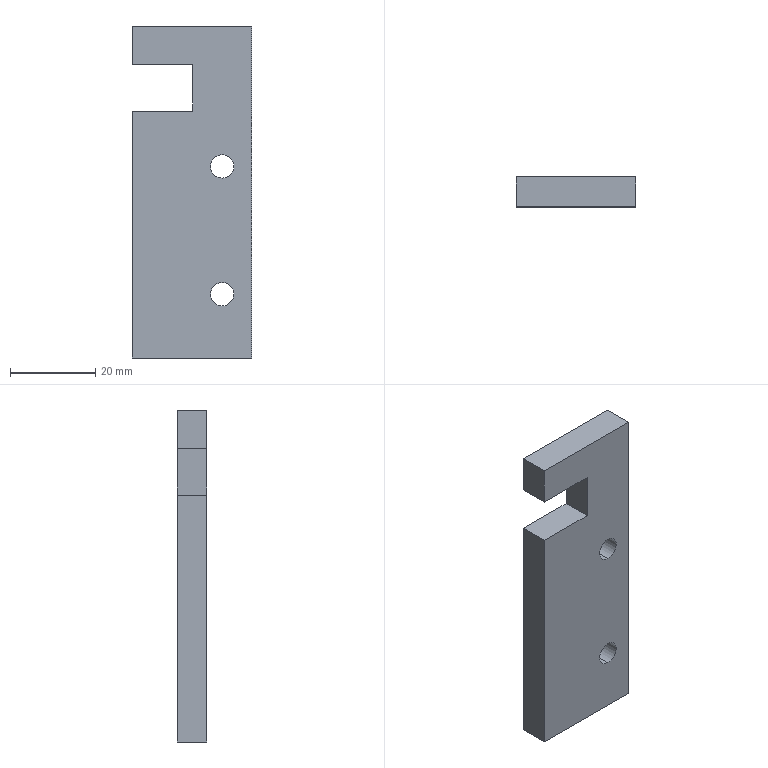Component | SolidWorks | PointedHeadDispensingCoverPlateA-1 | 1 solid | 14 faces | box 28 x 7 x 78 mm | volume 13862 mm3 | plane 10 | cylinder 4 | commonest cylinder face diameters 5.5 x4
build123d program:
from build123d import *

# Parameters (mm, degrees)
SKETCH1_W                  = 28
SKETCH1_H                  = 78
EXTRUDE1_DEPTH             = 7
SKETCH2_W                  = 14.2
SKETCH2_H                  = 11
CUT_EXTRUDE1_DEPTH         = 84.169
F_5_5_5_5_DIAMETER_HOLE1_D = 5.5


with BuildPart() as part:
    # Sketch1 → Extrude1 (new body)
    with BuildSketch(Plane(origin=(0, 0, 0), x_dir=(1, 0, 0), z_dir=(0, 1, 0))):
        with Locations((14, -39)):
            Rectangle(SKETCH1_W, SKETCH1_H)
    extrude(amount=EXTRUDE1_DEPTH)

    # Sketch2 → Cut-Extrude1 (cut, through all)
    with BuildSketch(Plane(origin=(0, 7, 0), x_dir=(1, 0, 0), z_dir=(0, 1, 0))):
        with Locations((7.1, -63.5)):
            Rectangle(SKETCH2_W, SKETCH2_H)
    extrude(amount=-CUT_EXTRUDE1_DEPTH, mode=Mode.SUBTRACT)

    # 5.5 _5.5_ Diameter Hole1 (through all)
    with Locations(Plane(origin=(0, 7, 0), x_dir=(-1, 0, 0), z_dir=(0, 1, 0))):
        with Locations((-21.1, 45), (-21.1, 15)):
            Hole(F_5_5_5_5_DIAMETER_HOLE1_D / 2)


solid = part.part

# Placed as in the assembly
solid = solid.moved(Location((10.917, 82.372, -117.387), (0, 0, 0)))
STEP:
#1=COLOUR_RGB('',0.7922,0.8196,0.9333);
#2=FILL_AREA_STYLE_COLOUR('',#1);
#3=FILL_AREA_STYLE('',(#2));
#4=SURFACE_STYLE_FILL_AREA(#3);
#5=SURFACE_SIDE_STYLE('',(#4));
#6=SURFACE_STYLE_USAGE(.BOTH.,#5);
#7=PRESENTATION_STYLE_ASSIGNMENT((#6));
#8=CARTESIAN_POINT('',(1.261,3.243,-2.958));
#9=VERTEX_POINT('',#8);
#10=CARTESIAN_POINT('',(1.261,3.243,-2.742));
#11=VERTEX_POINT('',#10);
#12=CARTESIAN_POINT('',(1.261,3.243,-2.85));
#13=DIRECTION('',(0.,1.,0.));
#14=DIRECTION('',(0.,0.,1.));
#15=AXIS2_PLACEMENT_3D('',#12,#13,#14);
#16=CIRCLE('',#15,0.1083);
#17=EDGE_CURVE('',#9,#11,#16,.T.);
#18=ORIENTED_EDGE('',*,*,#17,.F.);
#19=CARTESIAN_POINT('',(1.261,3.519,-2.958));
#20=VERTEX_POINT('',#19);
#21=CARTESIAN_POINT('',(1.261,3.519,-2.958));
#22=DIRECTION('',(0.,1.,0.));
#23=VECTOR('',#22,39.37);
#24=LINE('',#21,#23);
#25=EDGE_CURVE('',#9,#20,#24,.T.);
#26=ORIENTED_EDGE('',*,*,#25,.T.);
#27=CARTESIAN_POINT('',(1.261,3.519,-2.742));
#28=VERTEX_POINT('',#27);
#29=CARTESIAN_POINT('',(1.261,3.519,-2.85));
#30=DIRECTION('',(0.,1.,0.));
#31=DIRECTION('',(0.,0.,1.));
#32=AXIS2_PLACEMENT_3D('',#29,#30,#31);
#33=CIRCLE('',#32,0.1083);
#34=EDGE_CURVE('',#20,#28,#33,.T.);
#35=ORIENTED_EDGE('',*,*,#34,.T.);
#36=CARTESIAN_POINT('',(1.261,3.519,-2.742));
#37=DIRECTION('',(0.,1.,0.));
#38=VECTOR('',#37,39.37);
#39=LINE('',#36,#38);
#40=EDGE_CURVE('',#11,#28,#39,.T.);
#41=ORIENTED_EDGE('',*,*,#40,.F.);
#42=EDGE_LOOP('',(#18,#26,#35,#41));
#43=FACE_OUTER_BOUND('',#42,.T.);
#44=CARTESIAN_POINT('',(1.261,3.519,-2.85));
#45=DIRECTION('',(0.,1.,0.));
#46=DIRECTION('',(0.,0.,1.));
#47=AXIS2_PLACEMENT_3D('',#44,#45,#46);
#48=CYLINDRICAL_SURFACE('',#47,0.1083);
#49=ADVANCED_FACE('',(#43),#48,.F.);
#50=CARTESIAN_POINT('',(1.261,3.243,-4.139));
#51=VERTEX_POINT('',#50);
#52=CARTESIAN_POINT('',(1.261,3.243,-3.923));
#53=VERTEX_POINT('',#52);
#54=CARTESIAN_POINT('',(1.261,3.243,-4.031));
#55=DIRECTION('',(0.,1.,0.));
#56=DIRECTION('',(0.,0.,1.));
#57=AXIS2_PLACEMENT_3D('',#54,#55,#56);
#58=CIRCLE('',#57,0.1083);
#59=EDGE_CURVE('',#51,#53,#58,.T.);
#60=ORIENTED_EDGE('',*,*,#59,.F.);
#61=CARTESIAN_POINT('',(1.261,3.519,-4.139));
#62=VERTEX_POINT('',#61);
#63=CARTESIAN_POINT('',(1.261,3.519,-4.139));
#64=DIRECTION('',(0.,1.,0.));
#65=VECTOR('',#64,39.37);
#66=LINE('',#63,#65);
#67=EDGE_CURVE('',#51,#62,#66,.T.);
#68=ORIENTED_EDGE('',*,*,#67,.T.);
#69=CARTESIAN_POINT('',(1.261,3.519,-3.923));
#70=VERTEX_POINT('',#69);
#71=CARTESIAN_POINT('',(1.261,3.519,-4.031));
#72=DIRECTION('',(0.,1.,0.));
#73=DIRECTION('',(0.,0.,1.));
#74=AXIS2_PLACEMENT_3D('',#71,#72,#73);
#75=CIRCLE('',#74,0.1083);
#76=EDGE_CURVE('',#62,#70,#75,.T.);
#77=ORIENTED_EDGE('',*,*,#76,.T.);
#78=CARTESIAN_POINT('',(1.261,3.519,-3.923));
#79=DIRECTION('',(0.,1.,0.));
#80=VECTOR('',#79,39.37);
#81=LINE('',#78,#80);
#82=EDGE_CURVE('',#53,#70,#81,.T.);
#83=ORIENTED_EDGE('',*,*,#82,.F.);
#84=EDGE_LOOP('',(#60,#68,#77,#83));
#85=FACE_OUTER_BOUND('',#84,.T.);
#86=CARTESIAN_POINT('',(1.261,3.519,-4.031));
#87=DIRECTION('',(0.,1.,0.));
#88=DIRECTION('',(0.,0.,1.));
#89=AXIS2_PLACEMENT_3D('',#86,#87,#88);
#90=CYLINDRICAL_SURFACE('',#89,0.1083);
#91=ADVANCED_FACE('',(#85),#90,.F.);
#92=CARTESIAN_POINT('',(0.4298,3.243,-4.622));
#93=VERTEX_POINT('',#92);
#94=CARTESIAN_POINT('',(0.4298,3.243,-2.338));
#95=VERTEX_POINT('',#94);
#96=CARTESIAN_POINT('',(0.4298,3.243,-4.622));
#97=DIRECTION('',(0.,0.,1.));
#98=VECTOR('',#97,39.37);
#99=LINE('',#96,#98);
#100=EDGE_CURVE('',#93,#95,#99,.T.);
#101=ORIENTED_EDGE('',*,*,#100,.T.);
#102=CARTESIAN_POINT('',(0.4298,3.519,-2.338));
#103=VERTEX_POINT('',#102);
#104=CARTESIAN_POINT('',(0.4298,3.243,-2.338));
#105=DIRECTION('',(0.,1.,0.));
#106=VECTOR('',#105,39.37);
#107=LINE('',#104,#106);
#108=EDGE_CURVE('',#95,#103,#107,.T.);
#109=ORIENTED_EDGE('',*,*,#108,.T.);
#110=CARTESIAN_POINT('',(0.4298,3.519,-4.622));
#111=VERTEX_POINT('',#110);
#112=CARTESIAN_POINT('',(0.4298,3.519,-4.622));
#113=DIRECTION('',(0.,0.,1.));
#114=VECTOR('',#113,39.37);
#115=LINE('',#112,#114);
#116=EDGE_CURVE('',#111,#103,#115,.T.);
#117=ORIENTED_EDGE('',*,*,#116,.F.);
#118=CARTESIAN_POINT('',(0.4298,3.519,-4.622));
#119=DIRECTION('',(0.,-1.,0.));
#120=VECTOR('',#119,39.37);
#121=LINE('',#118,#120);
#122=EDGE_CURVE('',#111,#93,#121,.T.);
#123=ORIENTED_EDGE('',*,*,#122,.T.);
#124=EDGE_LOOP('',(#101,#109,#117,#123));
#125=FACE_OUTER_BOUND('',#124,.T.);
#126=CARTESIAN_POINT('',(0.4298,3.519,-4.622));
#127=DIRECTION('',(1.,0.,-0.));
#128=DIRECTION('',(-0.,0.,-1.));
#129=AXIS2_PLACEMENT_3D('',#126,#127,#128);
#130=PLANE('',#129);
#131=ADVANCED_FACE('',(#125),#130,.F.);
#132=CARTESIAN_POINT('',(0.4298,3.519,-1.905));
#133=VERTEX_POINT('',#132);
#134=CARTESIAN_POINT('',(0.4298,3.519,-1.551));
#135=VERTEX_POINT('',#134);
#136=CARTESIAN_POINT('',(0.4298,3.519,-4.622));
#137=DIRECTION('',(0.,0.,1.));
#138=VECTOR('',#137,39.37);
#139=LINE('',#136,#138);
#140=EDGE_CURVE('',#133,#135,#139,.T.);
#141=ORIENTED_EDGE('',*,*,#140,.F.);
#142=CARTESIAN_POINT('',(0.4298,3.243,-1.905));
#143=VERTEX_POINT('',#142);
#144=CARTESIAN_POINT('',(0.4298,3.243,-1.905));
#145=DIRECTION('',(0.,1.,0.));
#146=VECTOR('',#145,39.37);
#147=LINE('',#144,#146);
#148=EDGE_CURVE('',#143,#133,#147,.T.);
#149=ORIENTED_EDGE('',*,*,#148,.F.);
#150=CARTESIAN_POINT('',(0.4298,3.243,-1.551));
#151=VERTEX_POINT('',#150);
#152=CARTESIAN_POINT('',(0.4298,3.243,-4.622));
#153=DIRECTION('',(0.,0.,1.));
#154=VECTOR('',#153,39.37);
#155=LINE('',#152,#154);
#156=EDGE_CURVE('',#143,#151,#155,.T.);
#157=ORIENTED_EDGE('',*,*,#156,.T.);
#158=CARTESIAN_POINT('',(0.4298,3.519,-1.551));
#159=DIRECTION('',(0.,-1.,0.));
#160=VECTOR('',#159,39.37);
#161=LINE('',#158,#160);
#162=EDGE_CURVE('',#135,#151,#161,.T.);
#163=ORIENTED_EDGE('',*,*,#162,.F.);
#164=EDGE_LOOP('',(#141,#149,#157,#163));
#165=FACE_OUTER_BOUND('',#164,.T.);
#166=CARTESIAN_POINT('',(0.4298,3.519,-4.622));
#167=DIRECTION('',(1.,0.,-0.));
#168=DIRECTION('',(-0.,0.,-1.));
#169=AXIS2_PLACEMENT_3D('',#166,#167,#168);
#170=PLANE('',#169);
#171=ADVANCED_FACE('',(#165),#170,.F.);
#172=CARTESIAN_POINT('',(1.532,3.243,-1.551));
#173=VERTEX_POINT('',#172);
#174=CARTESIAN_POINT('',(0.4298,3.243,-1.551));
#175=DIRECTION('',(1.,0.,0.));
#176=VECTOR('',#175,39.37);
#177=LINE('',#174,#176);
#178=EDGE_CURVE('',#151,#173,#177,.T.);
#179=ORIENTED_EDGE('',*,*,#178,.T.);
#180=CARTESIAN_POINT('',(1.532,3.519,-1.551));
#181=VERTEX_POINT('',#180);
#182=CARTESIAN_POINT('',(1.532,3.519,-1.551));
#183=DIRECTION('',(0.,-1.,0.));
#184=VECTOR('',#183,39.37);
#185=LINE('',#182,#184);
#186=EDGE_CURVE('',#181,#173,#185,.T.);
#187=ORIENTED_EDGE('',*,*,#186,.F.);
#188=CARTESIAN_POINT('',(0.4298,3.519,-1.551));
#189=DIRECTION('',(1.,0.,0.));
#190=VECTOR('',#189,39.37);
#191=LINE('',#188,#190);
#192=EDGE_CURVE('',#135,#181,#191,.T.);
#193=ORIENTED_EDGE('',*,*,#192,.F.);
#194=ORIENTED_EDGE('',*,*,#162,.T.);
#195=EDGE_LOOP('',(#179,#187,#193,#194));
#196=FACE_OUTER_BOUND('',#195,.T.);
#197=CARTESIAN_POINT('',(0.4298,3.519,-1.551));
#198=DIRECTION('',(0.,0.,-1.));
#199=DIRECTION('',(-1.,0.,0.));
#200=AXIS2_PLACEMENT_3D('',#197,#198,#199);
#201=PLANE('',#200);
#202=ADVANCED_FACE('',(#196),#201,.F.);
#203=CARTESIAN_POINT('',(1.532,3.243,-4.622));
#204=VERTEX_POINT('',#203);
#205=CARTESIAN_POINT('',(1.532,3.243,-4.622));
#206=DIRECTION('',(-0.,0.,-1.));
#207=VECTOR('',#206,39.37);
#208=LINE('',#205,#207);
#209=EDGE_CURVE('',#173,#204,#208,.T.);
#210=ORIENTED_EDGE('',*,*,#209,.T.);
#211=CARTESIAN_POINT('',(1.532,3.519,-4.622));
#212=VERTEX_POINT('',#211);
#213=CARTESIAN_POINT('',(1.532,3.519,-4.622));
#214=DIRECTION('',(0.,-1.,0.));
#215=VECTOR('',#214,39.37);
#216=LINE('',#213,#215);
#217=EDGE_CURVE('',#212,#204,#216,.T.);
#218=ORIENTED_EDGE('',*,*,#217,.F.);
#219=CARTESIAN_POINT('',(1.532,3.519,-4.622));
#220=DIRECTION('',(-0.,0.,-1.));
#221=VECTOR('',#220,39.37);
#222=LINE('',#219,#221);
#223=EDGE_CURVE('',#181,#212,#222,.T.);
#224=ORIENTED_EDGE('',*,*,#223,.F.);
#225=ORIENTED_EDGE('',*,*,#186,.T.);
#226=EDGE_LOOP('',(#210,#218,#224,#225));
#227=FACE_OUTER_BOUND('',#226,.T.);
#228=CARTESIAN_POINT('',(1.532,3.519,-4.622));
#229=DIRECTION('',(-1.,0.,0.));
#230=DIRECTION('',(0.,0.,1.));
#231=AXIS2_PLACEMENT_3D('',#228,#229,#230);
#232=PLANE('',#231);
#233=ADVANCED_FACE('',(#227),#232,.F.);
#234=CARTESIAN_POINT('',(0.4298,3.243,-4.622));
#235=DIRECTION('',(-1.,0.,0.));
#236=VECTOR('',#235,39.37);
#237=LINE('',#234,#236);
#238=EDGE_CURVE('',#204,#93,#237,.T.);
#239=ORIENTED_EDGE('',*,*,#238,.T.);
#240=ORIENTED_EDGE('',*,*,#122,.F.);
#241=CARTESIAN_POINT('',(0.4298,3.519,-4.622));
#242=DIRECTION('',(-1.,0.,0.));
#243=VECTOR('',#242,39.37);
#244=LINE('',#241,#243);
#245=EDGE_CURVE('',#212,#111,#244,.T.);
#246=ORIENTED_EDGE('',*,*,#245,.F.);
#247=ORIENTED_EDGE('',*,*,#217,.T.);
#248=EDGE_LOOP('',(#239,#240,#246,#247));
#249=FACE_OUTER_BOUND('',#248,.T.);
#250=CARTESIAN_POINT('',(0.4298,3.519,-4.622));
#251=DIRECTION('',(0.,0.,1.));
#252=DIRECTION('',(1.,0.,0.));
#253=AXIS2_PLACEMENT_3D('',#250,#251,#252);
#254=PLANE('',#253);
#255=ADVANCED_FACE('',(#249),#254,.F.);
#256=CARTESIAN_POINT('',(1.261,3.519,-2.85));
#257=DIRECTION('',(0.,1.,0.));
#258=DIRECTION('',(0.,0.,1.));
#259=AXIS2_PLACEMENT_3D('',#256,#257,#258);
#260=CIRCLE('',#259,0.1083);
#261=EDGE_CURVE('',#28,#20,#260,.T.);
#262=ORIENTED_EDGE('',*,*,#261,.F.);
#263=ORIENTED_EDGE('',*,*,#34,.F.);
#264=EDGE_LOOP('',(#262,#263));
#265=FACE_BOUND('',#264,.T.);
#266=CARTESIAN_POINT('',(1.261,3.519,-4.031));
#267=DIRECTION('',(0.,1.,0.));
#268=DIRECTION('',(0.,0.,1.));
#269=AXIS2_PLACEMENT_3D('',#266,#267,#268);
#270=CIRCLE('',#269,0.1083);
#271=EDGE_CURVE('',#70,#62,#270,.T.);
#272=ORIENTED_EDGE('',*,*,#271,.F.);
#273=ORIENTED_EDGE('',*,*,#76,.F.);
#274=EDGE_LOOP('',(#272,#273));
#275=FACE_BOUND('',#274,.T.);
#276=CARTESIAN_POINT('',(0.9889,3.519,-2.338));
#277=VERTEX_POINT('',#276);
#278=CARTESIAN_POINT('',(0.4298,3.519,-2.338));
#279=DIRECTION('',(-1.,0.,-0.));
#280=VECTOR('',#279,39.37);
#281=LINE('',#278,#280);
#282=EDGE_CURVE('',#277,#103,#281,.T.);
#283=ORIENTED_EDGE('',*,*,#282,.F.);
#284=CARTESIAN_POINT('',(0.9889,3.519,-1.905));
#285=VERTEX_POINT('',#284);
#286=CARTESIAN_POINT('',(0.9889,3.519,-1.905));
#287=DIRECTION('',(0.,0.,-1.));
#288=VECTOR('',#287,39.37);
#289=LINE('',#286,#288);
#290=EDGE_CURVE('',#285,#277,#289,.T.);
#291=ORIENTED_EDGE('',*,*,#290,.F.);
#292=CARTESIAN_POINT('',(0.4298,3.519,-1.905));
#293=DIRECTION('',(1.,0.,0.));
#294=VECTOR('',#293,39.37);
#295=LINE('',#292,#294);
#296=EDGE_CURVE('',#133,#285,#295,.T.);
#297=ORIENTED_EDGE('',*,*,#296,.F.);
#298=ORIENTED_EDGE('',*,*,#140,.T.);
#299=ORIENTED_EDGE('',*,*,#192,.T.);
#300=ORIENTED_EDGE('',*,*,#223,.T.);
#301=ORIENTED_EDGE('',*,*,#245,.T.);
#302=ORIENTED_EDGE('',*,*,#116,.T.);
#303=EDGE_LOOP('',(#283,#291,#297,#298,#299,#300,#301,#302));
#304=FACE_OUTER_BOUND('',#303,.T.);
#305=CARTESIAN_POINT('',(0.4298,3.519,-1.551));
#306=DIRECTION('',(0.,1.,0.));
#307=DIRECTION('',(0.,0.,1.));
#308=AXIS2_PLACEMENT_3D('',#305,#306,#307);
#309=PLANE('',#308);
#310=ADVANCED_FACE('',(#265,#275,#304),#309,.T.);
#311=CARTESIAN_POINT('',(1.261,3.243,-2.85));
#312=DIRECTION('',(0.,1.,0.));
#313=DIRECTION('',(0.,0.,1.));
#314=AXIS2_PLACEMENT_3D('',#311,#312,#313);
#315=CIRCLE('',#314,0.1083);
#316=EDGE_CURVE('',#11,#9,#315,.T.);
#317=ORIENTED_EDGE('',*,*,#316,.T.);
#318=ORIENTED_EDGE('',*,*,#17,.T.);
#319=EDGE_LOOP('',(#317,#318));
#320=FACE_BOUND('',#319,.T.);
#321=CARTESIAN_POINT('',(1.261,3.243,-4.031));
#322=DIRECTION('',(0.,1.,0.));
#323=DIRECTION('',(0.,0.,1.));
#324=AXIS2_PLACEMENT_3D('',#321,#322,#323);
#325=CIRCLE('',#324,0.1083);
#326=EDGE_CURVE('',#53,#51,#325,.T.);
#327=ORIENTED_EDGE('',*,*,#326,.T.);
#328=ORIENTED_EDGE('',*,*,#59,.T.);
#329=EDGE_LOOP('',(#327,#328));
#330=FACE_BOUND('',#329,.T.);
#331=CARTESIAN_POINT('',(0.9889,3.243,-1.905));
#332=VERTEX_POINT('',#331);
#333=CARTESIAN_POINT('',(0.9889,3.243,-2.338));
#334=VERTEX_POINT('',#333);
#335=CARTESIAN_POINT('',(0.9889,3.243,-1.905));
#336=DIRECTION('',(0.,0.,-1.));
#337=VECTOR('',#336,39.37);
#338=LINE('',#335,#337);
#339=EDGE_CURVE('',#332,#334,#338,.T.);
#340=ORIENTED_EDGE('',*,*,#339,.T.);
#341=CARTESIAN_POINT('',(0.4298,3.243,-2.338));
#342=DIRECTION('',(-1.,0.,-0.));
#343=VECTOR('',#342,39.37);
#344=LINE('',#341,#343);
#345=EDGE_CURVE('',#334,#95,#344,.T.);
#346=ORIENTED_EDGE('',*,*,#345,.T.);
#347=ORIENTED_EDGE('',*,*,#100,.F.);
#348=ORIENTED_EDGE('',*,*,#238,.F.);
#349=ORIENTED_EDGE('',*,*,#209,.F.);
#350=ORIENTED_EDGE('',*,*,#178,.F.);
#351=ORIENTED_EDGE('',*,*,#156,.F.);
#352=CARTESIAN_POINT('',(0.4298,3.243,-1.905));
#353=DIRECTION('',(1.,0.,0.));
#354=VECTOR('',#353,39.37);
#355=LINE('',#352,#354);
#356=EDGE_CURVE('',#143,#332,#355,.T.);
#357=ORIENTED_EDGE('',*,*,#356,.T.);
#358=EDGE_LOOP('',(#340,#346,#347,#348,#349,#350,#351,#357));
#359=FACE_OUTER_BOUND('',#358,.T.);
#360=CARTESIAN_POINT('',(0.4298,3.243,-1.551));
#361=DIRECTION('',(0.,1.,0.));
#362=DIRECTION('',(0.,0.,1.));
#363=AXIS2_PLACEMENT_3D('',#360,#361,#362);
#364=PLANE('',#363);
#365=ADVANCED_FACE('',(#320,#330,#359),#364,.F.);
#366=ORIENTED_EDGE('',*,*,#282,.T.);
#367=ORIENTED_EDGE('',*,*,#108,.F.);
#368=ORIENTED_EDGE('',*,*,#345,.F.);
#369=CARTESIAN_POINT('',(0.9889,3.243,-2.338));
#370=DIRECTION('',(0.,1.,0.));
#371=VECTOR('',#370,39.37);
#372=LINE('',#369,#371);
#373=EDGE_CURVE('',#334,#277,#372,.T.);
#374=ORIENTED_EDGE('',*,*,#373,.T.);
#375=EDGE_LOOP('',(#366,#367,#368,#374));
#376=FACE_OUTER_BOUND('',#375,.T.);
#377=CARTESIAN_POINT('',(0.4298,3.243,-2.338));
#378=DIRECTION('',(0.,0.,-1.));
#379=DIRECTION('',(-1.,0.,-0.));
#380=AXIS2_PLACEMENT_3D('',#377,#378,#379);
#381=PLANE('',#380);
#382=ADVANCED_FACE('',(#376),#381,.F.);
#383=ORIENTED_EDGE('',*,*,#290,.T.);
#384=ORIENTED_EDGE('',*,*,#373,.F.);
#385=ORIENTED_EDGE('',*,*,#339,.F.);
#386=CARTESIAN_POINT('',(0.9889,3.243,-1.905));
#387=DIRECTION('',(0.,1.,0.));
#388=VECTOR('',#387,39.37);
#389=LINE('',#386,#388);
#390=EDGE_CURVE('',#332,#285,#389,.T.);
#391=ORIENTED_EDGE('',*,*,#390,.T.);
#392=EDGE_LOOP('',(#383,#384,#385,#391));
#393=FACE_OUTER_BOUND('',#392,.T.);
#394=CARTESIAN_POINT('',(0.9889,3.243,-1.905));
#395=DIRECTION('',(1.,0.,0.));
#396=DIRECTION('',(0.,0.,-1.));
#397=AXIS2_PLACEMENT_3D('',#394,#395,#396);
#398=PLANE('',#397);
#399=ADVANCED_FACE('',(#393),#398,.F.);
#400=ORIENTED_EDGE('',*,*,#296,.T.);
#401=ORIENTED_EDGE('',*,*,#390,.F.);
#402=ORIENTED_EDGE('',*,*,#356,.F.);
#403=ORIENTED_EDGE('',*,*,#148,.T.);
#404=EDGE_LOOP('',(#400,#401,#402,#403));
#405=FACE_OUTER_BOUND('',#404,.T.);
#406=CARTESIAN_POINT('',(0.4298,3.243,-1.905));
#407=DIRECTION('',(0.,0.,1.));
#408=DIRECTION('',(1.,0.,0.));
#409=AXIS2_PLACEMENT_3D('',#406,#407,#408);
#410=PLANE('',#409);
#411=ADVANCED_FACE('',(#405),#410,.F.);
#412=ORIENTED_EDGE('',*,*,#67,.F.);
#413=ORIENTED_EDGE('',*,*,#326,.F.);
#414=ORIENTED_EDGE('',*,*,#82,.T.);
#415=ORIENTED_EDGE('',*,*,#271,.T.);
#416=EDGE_LOOP('',(#412,#413,#414,#415));
#417=FACE_OUTER_BOUND('',#416,.T.);
#418=CARTESIAN_POINT('',(1.261,3.519,-4.031));
#419=DIRECTION('',(0.,1.,0.));
#420=DIRECTION('',(0.,0.,1.));
#421=AXIS2_PLACEMENT_3D('',#418,#419,#420);
#422=CYLINDRICAL_SURFACE('',#421,0.1083);
#423=ADVANCED_FACE('',(#417),#422,.F.);
#424=ORIENTED_EDGE('',*,*,#25,.F.);
#425=ORIENTED_EDGE('',*,*,#316,.F.);
#426=ORIENTED_EDGE('',*,*,#40,.T.);
#427=ORIENTED_EDGE('',*,*,#261,.T.);
#428=EDGE_LOOP('',(#424,#425,#426,#427));
#429=FACE_OUTER_BOUND('',#428,.T.);
#430=CARTESIAN_POINT('',(1.261,3.519,-2.85));
#431=DIRECTION('',(0.,1.,0.));
#432=DIRECTION('',(0.,0.,1.));
#433=AXIS2_PLACEMENT_3D('',#430,#431,#432);
#434=CYLINDRICAL_SURFACE('',#433,0.1083);
#435=ADVANCED_FACE('',(#429),#434,.F.);
#436=CLOSED_SHELL('',(#49,#91,#131,#171,#202,#233,#255,#310,#365,#382,#399,#411,#423,#435));
#437=MANIFOLD_SOLID_BREP('',#436);
#438=STYLED_ITEM('',(#7),#437);
#439=PRESENTATION_LAYER_ASSIGNMENT('','',(#438));
#440=CARTESIAN_POINT('',(0.,0.,0.));
#441=DIRECTION('',(0.,0.,1.));
#442=DIRECTION('',(1.,0.,0.));
#443=AXIS2_PLACEMENT_3D('',#440,#441,#442);
#444=(LENGTH_UNIT()NAMED_UNIT(*)SI_UNIT($,.METRE.));
#445=LENGTH_MEASURE_WITH_UNIT(LENGTH_MEASURE(0.0254),#444);
#446=DIMENSIONAL_EXPONENTS(1.,0.,0.,0.,0.,0.,0.);
#447=(CONVERSION_BASED_UNIT('',#445)LENGTH_UNIT()NAMED_UNIT(#446));
#448=UNCERTAINTY_MEASURE_WITH_UNIT(LENGTH_MEASURE(0.00001),#447,'','');
#449=(NAMED_UNIT(*)PLANE_ANGLE_UNIT()SI_UNIT($,.RADIAN.));
#450=(NAMED_UNIT(*)SI_UNIT($,.STERADIAN.)SOLID_ANGLE_UNIT());
#451=(GEOMETRIC_REPRESENTATION_CONTEXT(3)GLOBAL_UNCERTAINTY_ASSIGNED_CONTEXT((#448))GLOBAL_UNIT_ASSIGNED_CONTEXT((#447,#449,#450))REPRESENTATION_CONTEXT('',''));
#452=ADVANCED_BREP_SHAPE_REPRESENTATION('',(#437,#443),#451);
#453=(LENGTH_UNIT()NAMED_UNIT(*)SI_UNIT($,.METRE.));
#454=LENGTH_MEASURE_WITH_UNIT(LENGTH_MEASURE(0.0254),#453);
#455=DIMENSIONAL_EXPONENTS(1.,0.,0.,0.,0.,0.,0.);
#456=(CONVERSION_BASED_UNIT('',#454)LENGTH_UNIT()NAMED_UNIT(#455));
#457=UNCERTAINTY_MEASURE_WITH_UNIT(LENGTH_MEASURE(0.00001),#456,'','');
#458=(NAMED_UNIT(*)PLANE_ANGLE_UNIT()SI_UNIT($,.RADIAN.));
#459=(NAMED_UNIT(*)SI_UNIT($,.STERADIAN.)SOLID_ANGLE_UNIT());
#460=(GEOMETRIC_REPRESENTATION_CONTEXT(3)GLOBAL_UNCERTAINTY_ASSIGNED_CONTEXT((#457))GLOBAL_UNIT_ASSIGNED_CONTEXT((#456,#458,#459))REPRESENTATION_CONTEXT('',''));
#461=MECHANICAL_DESIGN_GEOMETRIC_PRESENTATION_REPRESENTATION('',(#438),#460);